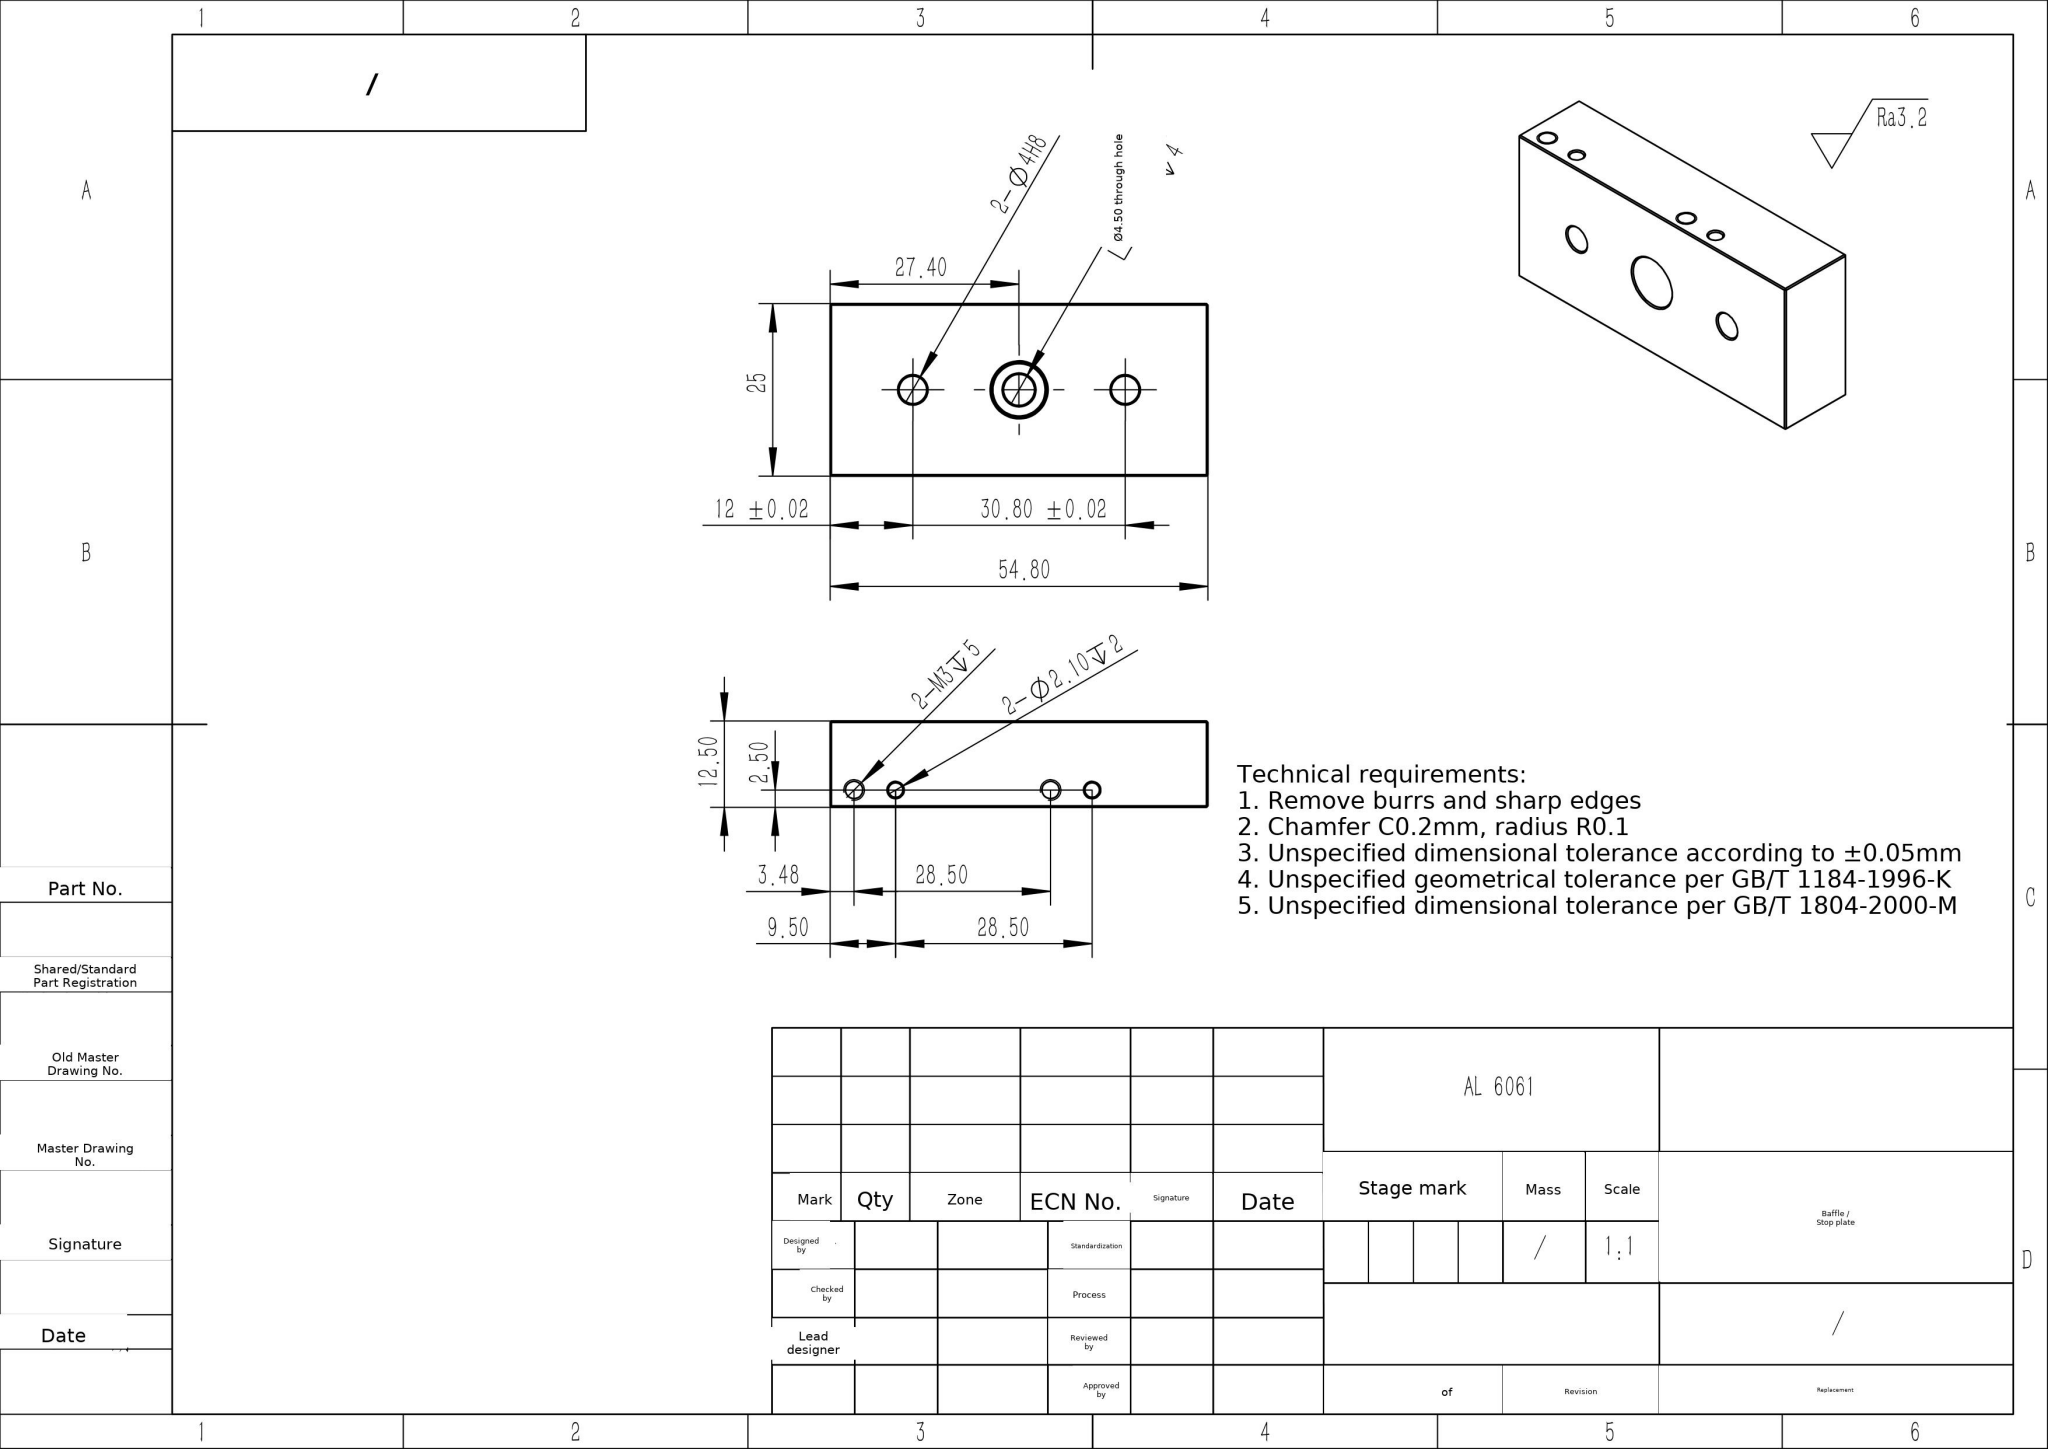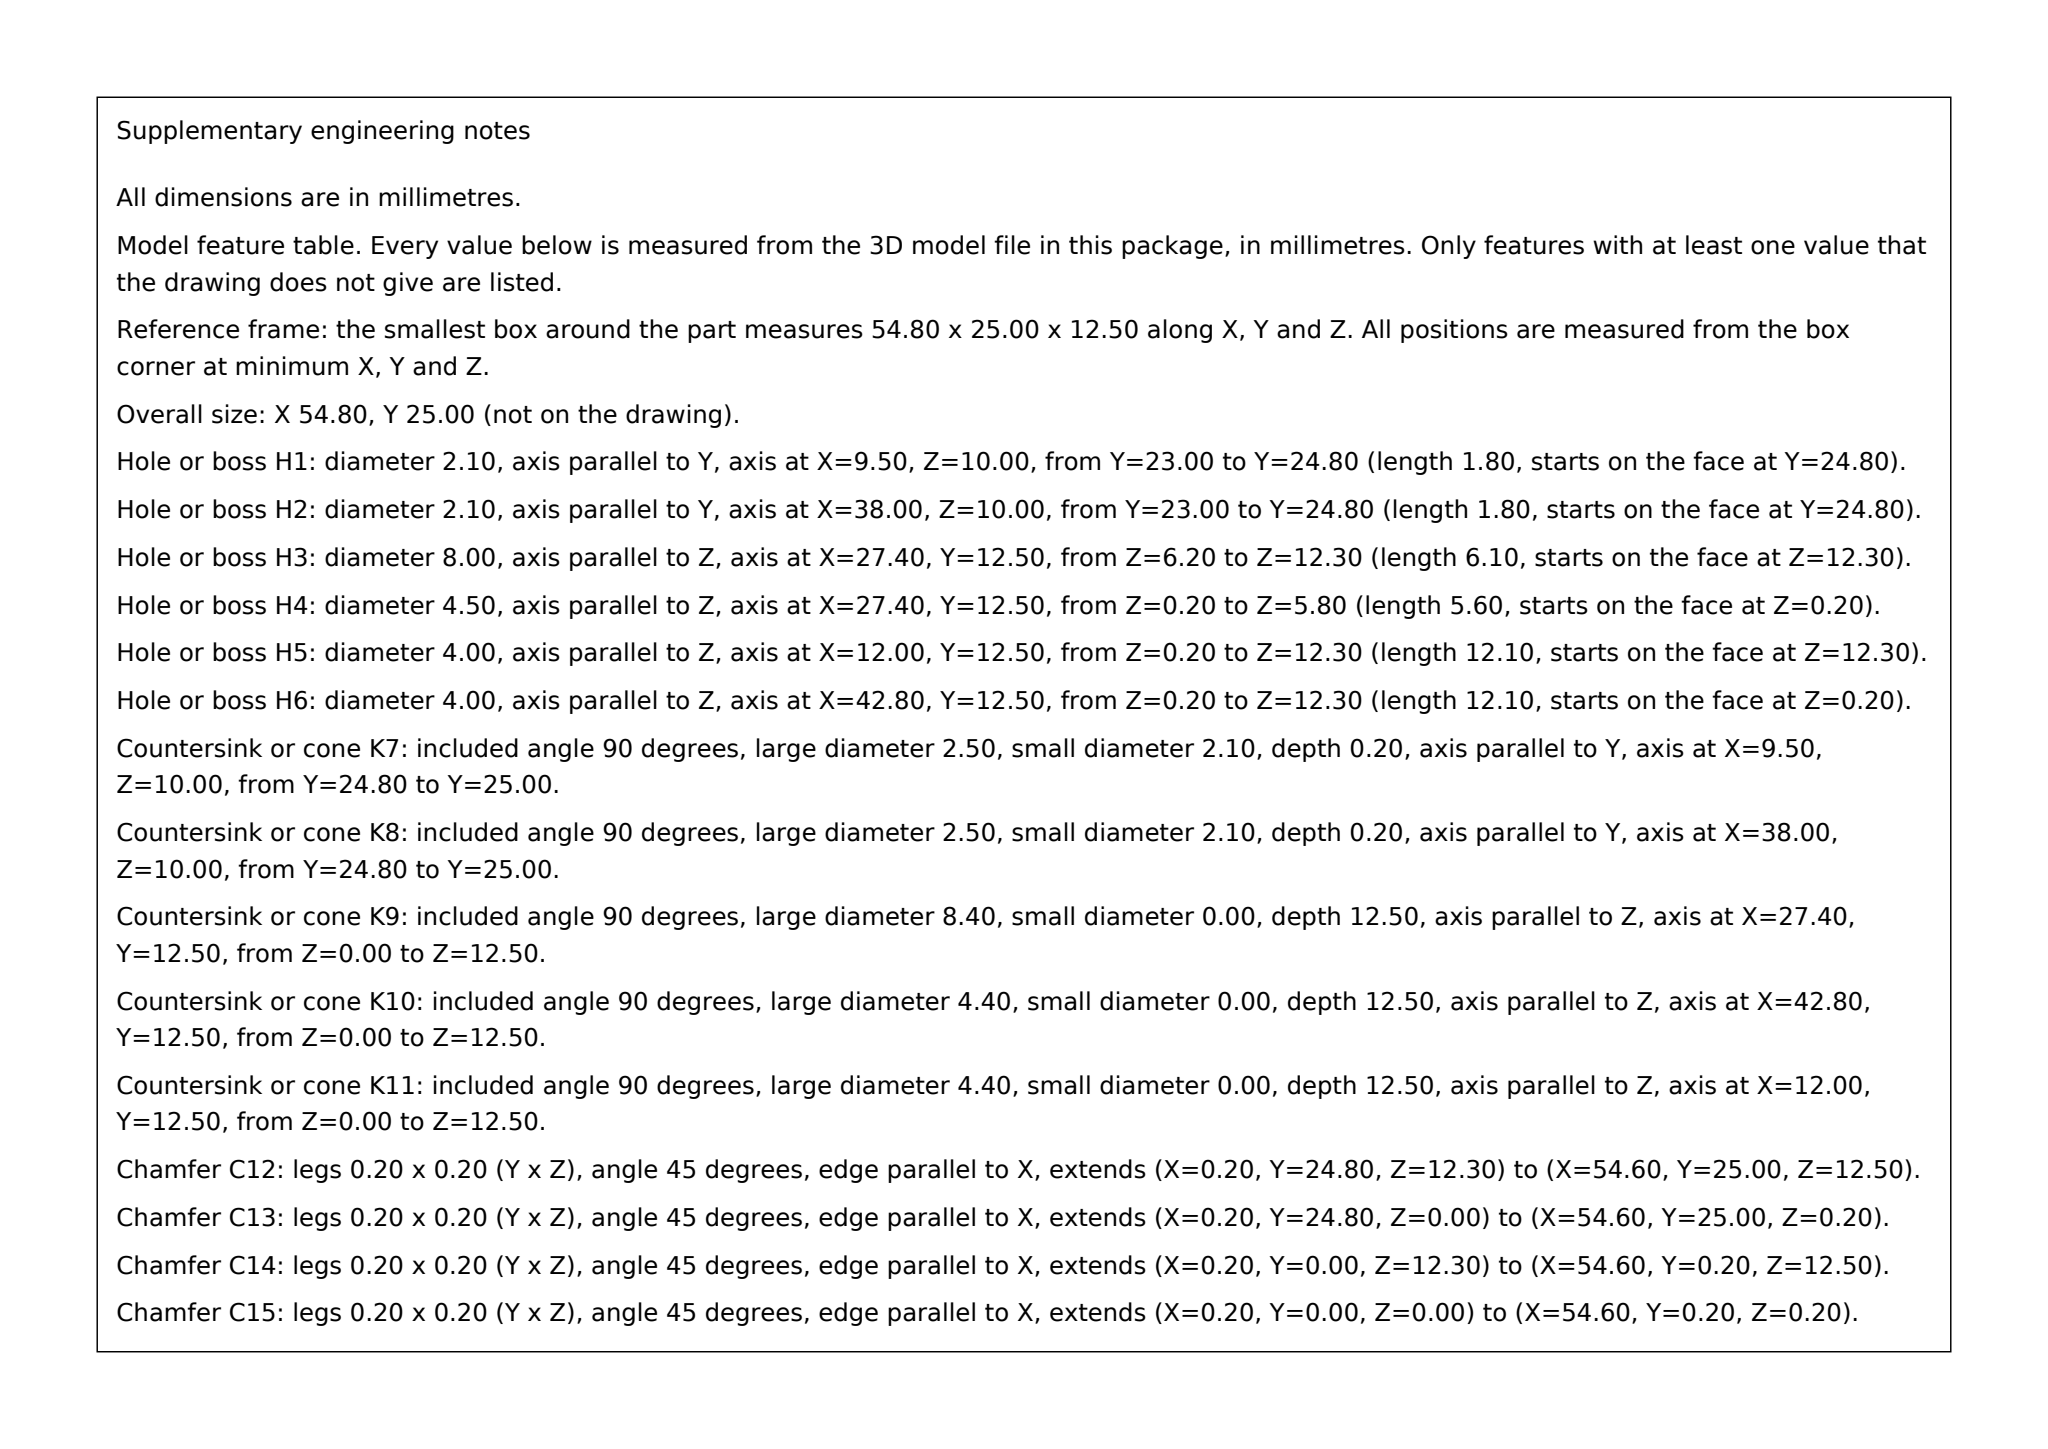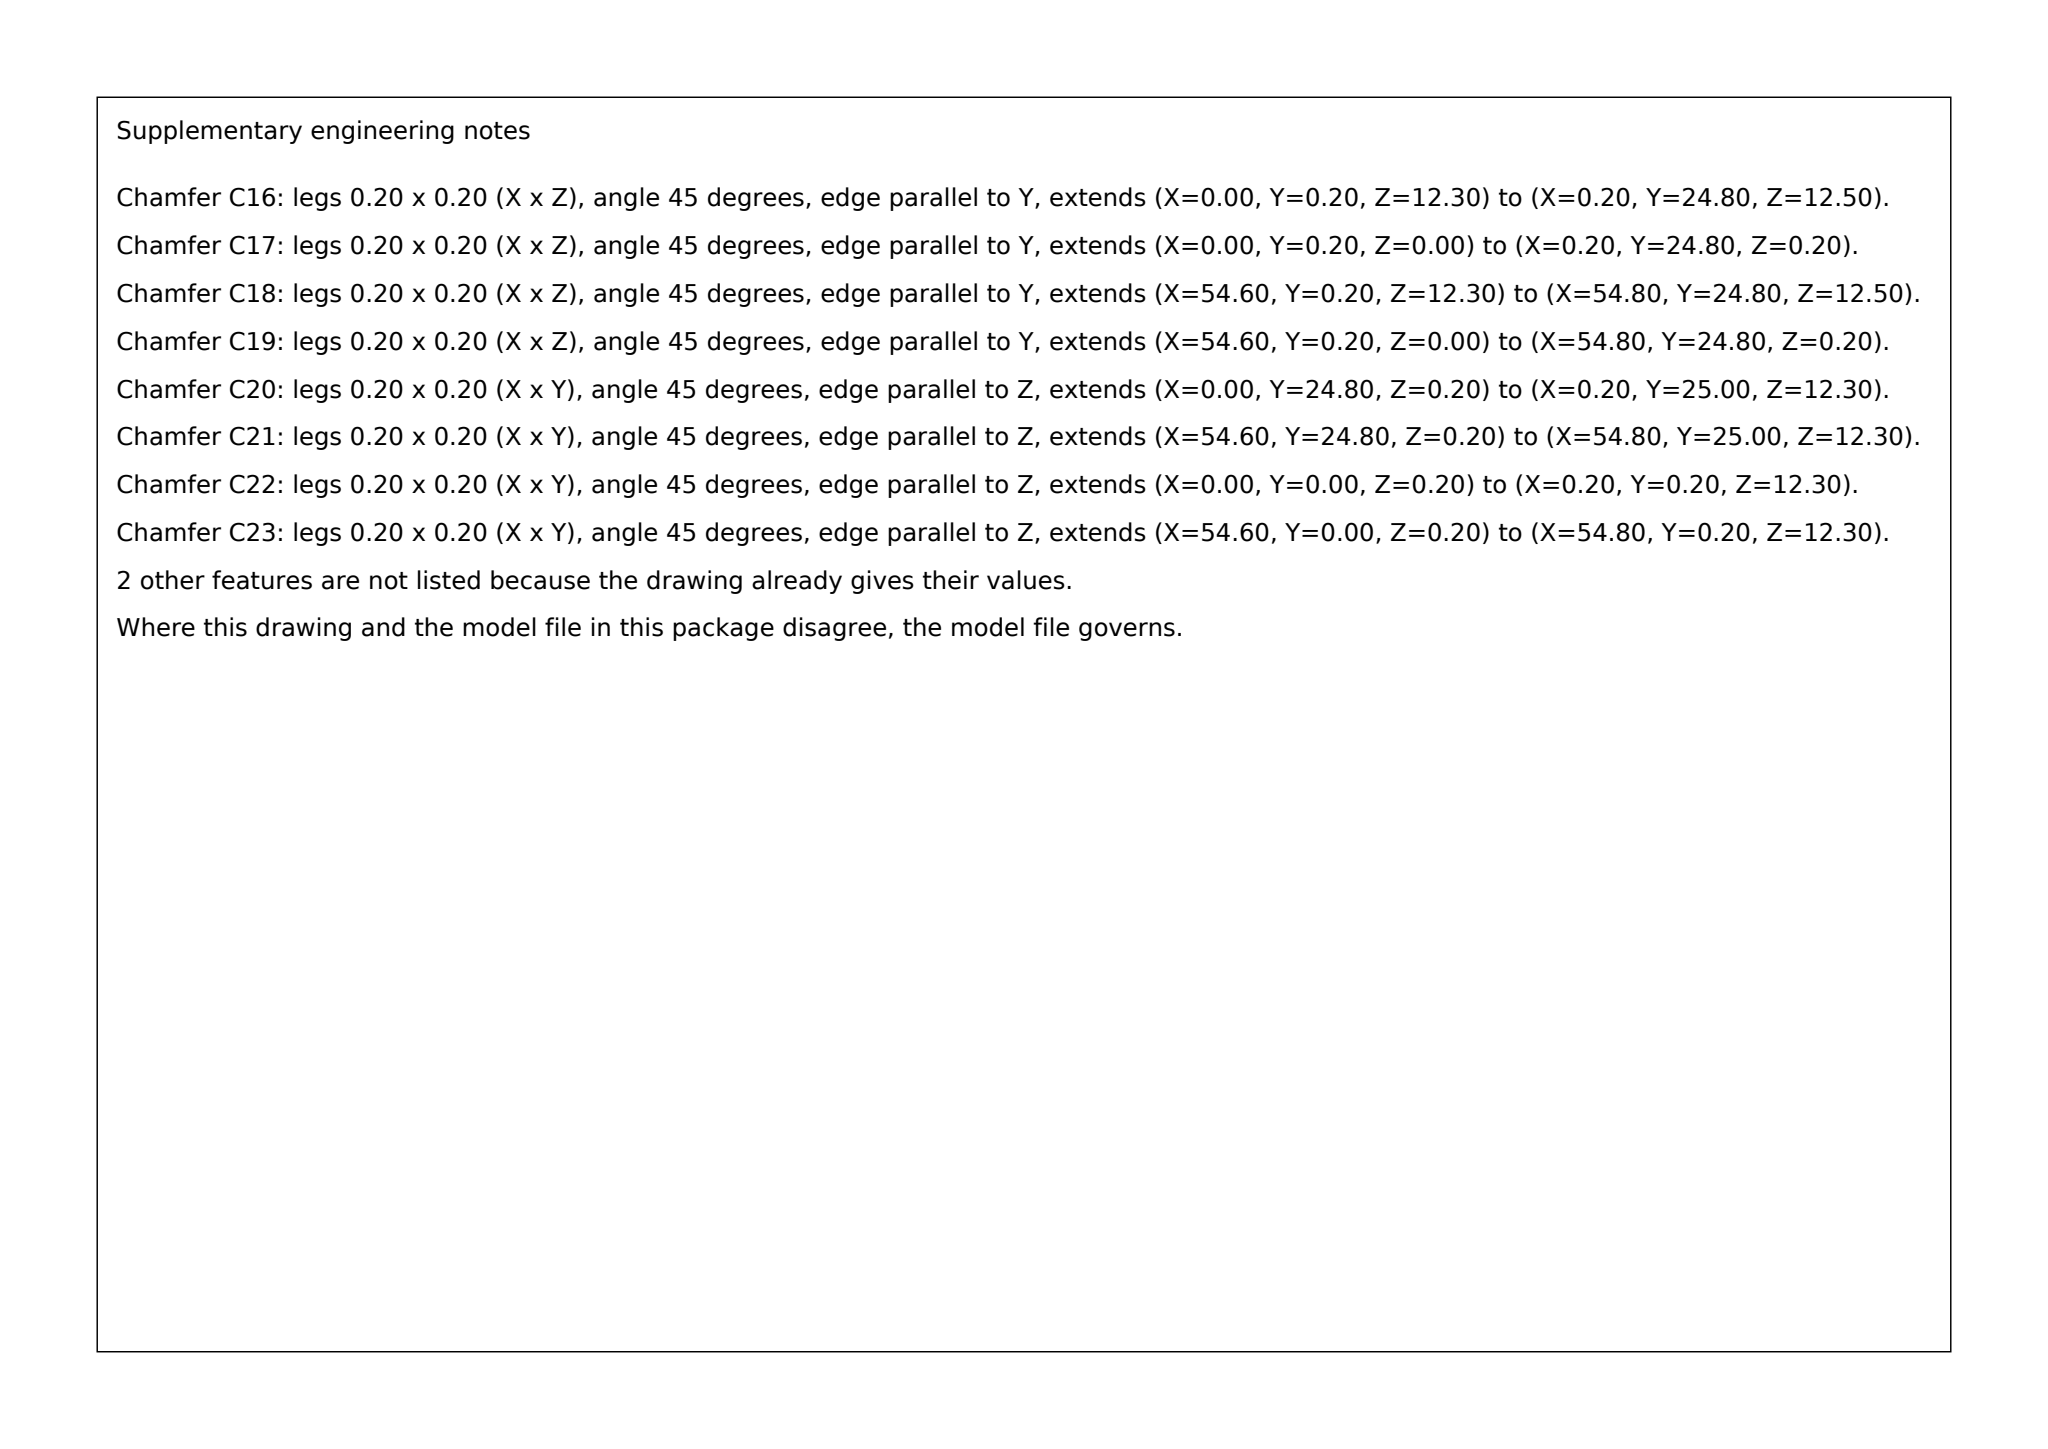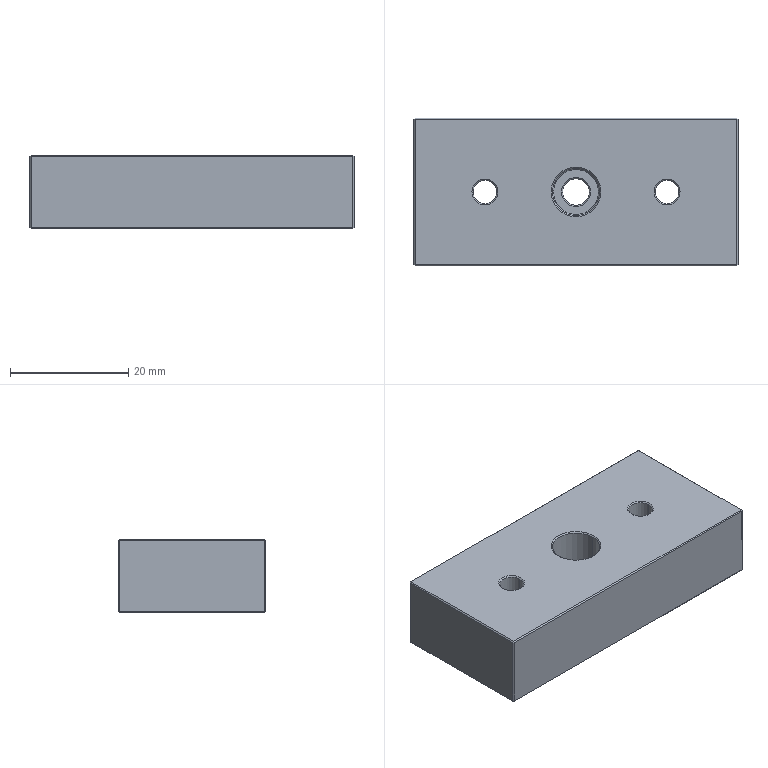Part | SolidWorks | mm | material AL 6061 | 1 solid | 69 faces | box 54.8 x 25 x 12.5 mm | volume 16309 mm3 | plane 29 | cone 24 | cylinder 16 | commonest cylinder face diameters 2.1 x4 2.5 x4 4 x4 4.5 x2 8 x2